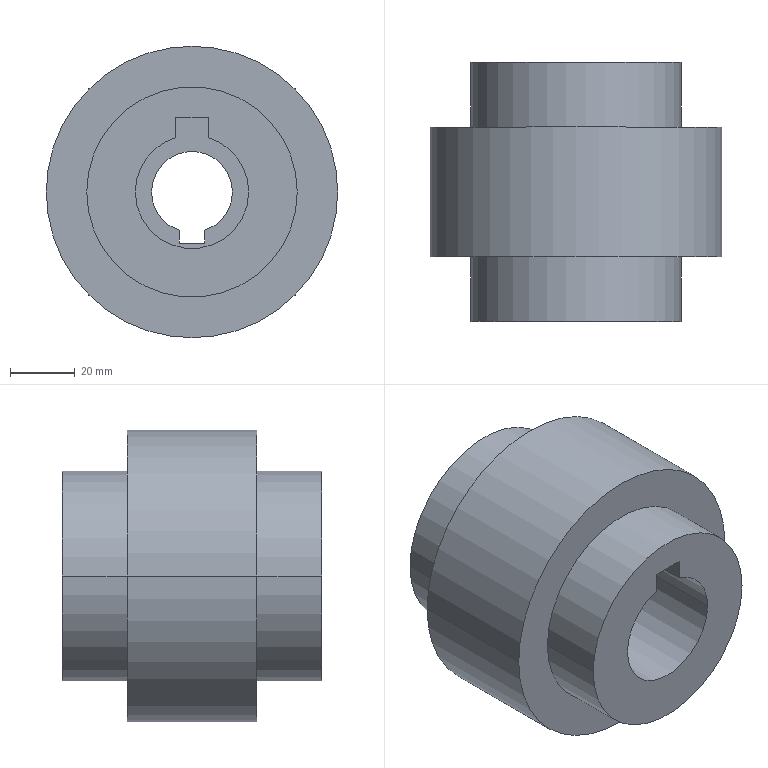Component | SolidWorks | TractorCoupling-1 | 1 solid | 23 faces | box 90 x 80 x 90 mm | volume 325660 mm3 | cylinder 12 | plane 11 | commonest cylinder face diameters 65 x4 35 x3 25 x3 90 x2
STEP:
#1=COLOUR_RGB('',0.7922,0.8196,0.9333);
#2=FILL_AREA_STYLE_COLOUR('',#1);
#3=FILL_AREA_STYLE('',(#2));
#4=SURFACE_STYLE_FILL_AREA(#3);
#5=SURFACE_SIDE_STYLE('',(#4));
#6=SURFACE_STYLE_USAGE(.BOTH.,#5);
#7=PRESENTATION_STYLE_ASSIGNMENT((#6));
#8=CARTESIAN_POINT('',(7.382,33.858,-6.811));
#9=VERTEX_POINT('',#8);
#10=CARTESIAN_POINT('',(8.76,33.858,-6.811));
#11=VERTEX_POINT('',#10);
#12=CARTESIAN_POINT('',(8.071,33.858,-6.811));
#13=DIRECTION('',(0.,-1.,0.));
#14=DIRECTION('',(1.,0.,0.));
#15=AXIS2_PLACEMENT_3D('',#12,#13,#14);
#16=CIRCLE('',#15,0.689);
#17=EDGE_CURVE('',#9,#11,#16,.T.);
#18=ORIENTED_EDGE('',*,*,#17,.F.);
#19=CARTESIAN_POINT('',(7.382,32.283,-6.811));
#20=VERTEX_POINT('',#19);
#21=CARTESIAN_POINT('',(7.382,33.858,-6.811));
#22=DIRECTION('',(0.,-1.,0.));
#23=VECTOR('',#22,39.37);
#24=LINE('',#21,#23);
#25=EDGE_CURVE('',#9,#20,#24,.T.);
#26=ORIENTED_EDGE('',*,*,#25,.T.);
#27=CARTESIAN_POINT('',(8.76,32.283,-6.811));
#28=VERTEX_POINT('',#27);
#29=CARTESIAN_POINT('',(8.071,32.283,-6.811));
#30=DIRECTION('',(0.,-1.,0.));
#31=DIRECTION('',(1.,0.,0.));
#32=AXIS2_PLACEMENT_3D('',#29,#30,#31);
#33=CIRCLE('',#32,0.689);
#34=EDGE_CURVE('',#20,#28,#33,.T.);
#35=ORIENTED_EDGE('',*,*,#34,.T.);
#36=CARTESIAN_POINT('',(8.76,33.858,-6.811));
#37=DIRECTION('',(0.,-1.,0.));
#38=VECTOR('',#37,39.37);
#39=LINE('',#36,#38);
#40=EDGE_CURVE('',#11,#28,#39,.T.);
#41=ORIENTED_EDGE('',*,*,#40,.F.);
#42=EDGE_LOOP('',(#18,#26,#35,#41));
#43=FACE_OUTER_BOUND('',#42,.T.);
#44=CARTESIAN_POINT('',(8.071,33.858,-6.811));
#45=DIRECTION('',(0.,-1.,0.));
#46=DIRECTION('',(1.,0.,0.));
#47=AXIS2_PLACEMENT_3D('',#44,#45,#46);
#48=CYLINDRICAL_SURFACE('',#47,0.689);
#49=ADVANCED_FACE('',(#43),#48,.F.);
#50=CARTESIAN_POINT('',(8.268,33.858,-6.151));
#51=VERTEX_POINT('',#50);
#52=CARTESIAN_POINT('',(8.071,33.858,-6.811));
#53=DIRECTION('',(0.,-1.,0.));
#54=DIRECTION('',(1.,0.,0.));
#55=AXIS2_PLACEMENT_3D('',#52,#53,#54);
#56=CIRCLE('',#55,0.689);
#57=EDGE_CURVE('',#11,#51,#56,.T.);
#58=ORIENTED_EDGE('',*,*,#57,.F.);
#59=ORIENTED_EDGE('',*,*,#40,.T.);
#60=CARTESIAN_POINT('',(8.268,32.283,-6.151));
#61=VERTEX_POINT('',#60);
#62=CARTESIAN_POINT('',(8.071,32.283,-6.811));
#63=DIRECTION('',(0.,-1.,0.));
#64=DIRECTION('',(1.,0.,0.));
#65=AXIS2_PLACEMENT_3D('',#62,#63,#64);
#66=CIRCLE('',#65,0.689);
#67=EDGE_CURVE('',#28,#61,#66,.T.);
#68=ORIENTED_EDGE('',*,*,#67,.T.);
#69=CARTESIAN_POINT('',(8.268,33.858,-6.151));
#70=DIRECTION('',(-0.,1.,0.));
#71=VECTOR('',#70,39.37);
#72=LINE('',#69,#71);
#73=EDGE_CURVE('',#61,#51,#72,.T.);
#74=ORIENTED_EDGE('',*,*,#73,.T.);
#75=EDGE_LOOP('',(#58,#59,#68,#74));
#76=FACE_OUTER_BOUND('',#75,.T.);
#77=CARTESIAN_POINT('',(8.071,33.858,-6.811));
#78=DIRECTION('',(0.,-1.,0.));
#79=DIRECTION('',(1.,0.,0.));
#80=AXIS2_PLACEMENT_3D('',#77,#78,#79);
#81=CYLINDRICAL_SURFACE('',#80,0.689);
#82=ADVANCED_FACE('',(#76),#81,.F.);
#83=CARTESIAN_POINT('',(6.791,32.283,-6.811));
#84=VERTEX_POINT('',#83);
#85=CARTESIAN_POINT('',(9.35,32.283,-6.811));
#86=VERTEX_POINT('',#85);
#87=CARTESIAN_POINT('',(8.071,32.283,-6.811));
#88=DIRECTION('',(0.,-1.,0.));
#89=DIRECTION('',(1.,0.,0.));
#90=AXIS2_PLACEMENT_3D('',#87,#88,#89);
#91=CIRCLE('',#90,1.28);
#92=EDGE_CURVE('',#84,#86,#91,.T.);
#93=ORIENTED_EDGE('',*,*,#92,.F.);
#94=CARTESIAN_POINT('',(6.791,33.071,-6.811));
#95=VERTEX_POINT('',#94);
#96=CARTESIAN_POINT('',(6.791,45.196,-6.811));
#97=DIRECTION('',(-0.,1.,0.));
#98=VECTOR('',#97,39.37);
#99=LINE('',#96,#98);
#100=EDGE_CURVE('',#84,#95,#99,.T.);
#101=ORIENTED_EDGE('',*,*,#100,.T.);
#102=CARTESIAN_POINT('',(9.35,33.071,-6.811));
#103=VERTEX_POINT('',#102);
#104=CARTESIAN_POINT('',(8.071,33.071,-6.811));
#105=DIRECTION('',(0.,-1.,0.));
#106=DIRECTION('',(1.,0.,0.));
#107=AXIS2_PLACEMENT_3D('',#104,#105,#106);
#108=CIRCLE('',#107,1.28);
#109=EDGE_CURVE('',#95,#103,#108,.T.);
#110=ORIENTED_EDGE('',*,*,#109,.T.);
#111=CARTESIAN_POINT('',(9.35,45.196,-6.811));
#112=DIRECTION('',(-0.,1.,0.));
#113=VECTOR('',#112,39.37);
#114=LINE('',#111,#113);
#115=EDGE_CURVE('',#86,#103,#114,.T.);
#116=ORIENTED_EDGE('',*,*,#115,.F.);
#117=EDGE_LOOP('',(#93,#101,#110,#116));
#118=FACE_OUTER_BOUND('',#117,.T.);
#119=CARTESIAN_POINT('',(8.071,45.196,-6.811));
#120=DIRECTION('',(-0.,1.,0.));
#121=DIRECTION('',(1.,0.,0.));
#122=AXIS2_PLACEMENT_3D('',#119,#120,#121);
#123=CYLINDRICAL_SURFACE('',#122,1.28);
#124=ADVANCED_FACE('',(#118),#123,.T.);
#125=CARTESIAN_POINT('',(9.35,35.433,-6.811));
#126=VERTEX_POINT('',#125);
#127=CARTESIAN_POINT('',(6.791,35.433,-6.811));
#128=VERTEX_POINT('',#127);
#129=CARTESIAN_POINT('',(8.071,35.433,-6.811));
#130=DIRECTION('',(0.,-1.,0.));
#131=DIRECTION('',(1.,0.,0.));
#132=AXIS2_PLACEMENT_3D('',#129,#130,#131);
#133=CIRCLE('',#132,1.28);
#134=EDGE_CURVE('',#126,#128,#133,.T.);
#135=ORIENTED_EDGE('',*,*,#134,.T.);
#136=CARTESIAN_POINT('',(6.791,34.646,-6.811));
#137=VERTEX_POINT('',#136);
#138=CARTESIAN_POINT('',(6.791,22.521,-6.811));
#139=DIRECTION('',(0.,-1.,0.));
#140=VECTOR('',#139,39.37);
#141=LINE('',#138,#140);
#142=EDGE_CURVE('',#128,#137,#141,.T.);
#143=ORIENTED_EDGE('',*,*,#142,.T.);
#144=CARTESIAN_POINT('',(9.35,34.646,-6.811));
#145=VERTEX_POINT('',#144);
#146=CARTESIAN_POINT('',(8.071,34.646,-6.811));
#147=DIRECTION('',(0.,-1.,0.));
#148=DIRECTION('',(1.,0.,0.));
#149=AXIS2_PLACEMENT_3D('',#146,#147,#148);
#150=CIRCLE('',#149,1.28);
#151=EDGE_CURVE('',#145,#137,#150,.T.);
#152=ORIENTED_EDGE('',*,*,#151,.F.);
#153=CARTESIAN_POINT('',(9.35,22.521,-6.811));
#154=DIRECTION('',(0.,-1.,0.));
#155=VECTOR('',#154,39.37);
#156=LINE('',#153,#155);
#157=EDGE_CURVE('',#126,#145,#156,.T.);
#158=ORIENTED_EDGE('',*,*,#157,.F.);
#159=EDGE_LOOP('',(#135,#143,#152,#158));
#160=FACE_OUTER_BOUND('',#159,.T.);
#161=CARTESIAN_POINT('',(8.071,22.521,-6.811));
#162=DIRECTION('',(0.,-1.,0.));
#163=DIRECTION('',(1.,0.,0.));
#164=AXIS2_PLACEMENT_3D('',#161,#162,#163);
#165=CYLINDRICAL_SURFACE('',#164,1.28);
#166=ADVANCED_FACE('',(#160),#165,.T.);
#167=CARTESIAN_POINT('',(9.843,34.646,-6.811));
#168=VERTEX_POINT('',#167);
#169=CARTESIAN_POINT('',(6.299,34.646,-6.811));
#170=VERTEX_POINT('',#169);
#171=CARTESIAN_POINT('',(8.071,34.646,-6.811));
#172=DIRECTION('',(0.,-1.,0.));
#173=DIRECTION('',(1.,0.,0.));
#174=AXIS2_PLACEMENT_3D('',#171,#172,#173);
#175=CIRCLE('',#174,1.772);
#176=EDGE_CURVE('',#168,#170,#175,.T.);
#177=ORIENTED_EDGE('',*,*,#176,.T.);
#178=CARTESIAN_POINT('',(6.299,33.071,-6.811));
#179=VERTEX_POINT('',#178);
#180=CARTESIAN_POINT('',(6.299,22.521,-6.811));
#181=DIRECTION('',(0.,-1.,0.));
#182=VECTOR('',#181,39.37);
#183=LINE('',#180,#182);
#184=EDGE_CURVE('',#170,#179,#183,.T.);
#185=ORIENTED_EDGE('',*,*,#184,.T.);
#186=CARTESIAN_POINT('',(9.843,33.071,-6.811));
#187=VERTEX_POINT('',#186);
#188=CARTESIAN_POINT('',(8.071,33.071,-6.811));
#189=DIRECTION('',(0.,-1.,0.));
#190=DIRECTION('',(1.,0.,0.));
#191=AXIS2_PLACEMENT_3D('',#188,#189,#190);
#192=CIRCLE('',#191,1.772);
#193=EDGE_CURVE('',#187,#179,#192,.T.);
#194=ORIENTED_EDGE('',*,*,#193,.F.);
#195=CARTESIAN_POINT('',(9.843,22.521,-6.811));
#196=DIRECTION('',(0.,-1.,0.));
#197=VECTOR('',#196,39.37);
#198=LINE('',#195,#197);
#199=EDGE_CURVE('',#168,#187,#198,.T.);
#200=ORIENTED_EDGE('',*,*,#199,.F.);
#201=EDGE_LOOP('',(#177,#185,#194,#200));
#202=FACE_OUTER_BOUND('',#201,.T.);
#203=CARTESIAN_POINT('',(8.071,22.521,-6.811));
#204=DIRECTION('',(0.,-1.,0.));
#205=DIRECTION('',(1.,0.,0.));
#206=AXIS2_PLACEMENT_3D('',#203,#204,#205);
#207=CYLINDRICAL_SURFACE('',#206,1.772);
#208=ADVANCED_FACE('',(#202),#207,.T.);
#209=CARTESIAN_POINT('',(7.579,35.433,-6.811));
#210=VERTEX_POINT('',#209);
#211=CARTESIAN_POINT('',(7.913,35.433,-7.277));
#212=VERTEX_POINT('',#211);
#213=CARTESIAN_POINT('',(8.071,35.433,-6.811));
#214=DIRECTION('',(0.,-1.,0.));
#215=DIRECTION('',(1.,0.,0.));
#216=AXIS2_PLACEMENT_3D('',#213,#214,#215);
#217=CIRCLE('',#216,0.4921);
#218=EDGE_CURVE('',#210,#212,#217,.T.);
#219=ORIENTED_EDGE('',*,*,#218,.F.);
#220=CARTESIAN_POINT('',(7.579,33.858,-6.811));
#221=VERTEX_POINT('',#220);
#222=CARTESIAN_POINT('',(7.579,22.521,-6.811));
#223=DIRECTION('',(0.,-1.,0.));
#224=VECTOR('',#223,39.37);
#225=LINE('',#222,#224);
#226=EDGE_CURVE('',#210,#221,#225,.T.);
#227=ORIENTED_EDGE('',*,*,#226,.T.);
#228=CARTESIAN_POINT('',(7.913,33.858,-7.277));
#229=VERTEX_POINT('',#228);
#230=CARTESIAN_POINT('',(8.071,33.858,-6.811));
#231=DIRECTION('',(0.,-1.,0.));
#232=DIRECTION('',(1.,0.,0.));
#233=AXIS2_PLACEMENT_3D('',#230,#231,#232);
#234=CIRCLE('',#233,0.4921);
#235=EDGE_CURVE('',#221,#229,#234,.T.);
#236=ORIENTED_EDGE('',*,*,#235,.T.);
#237=CARTESIAN_POINT('',(7.913,22.521,-7.277));
#238=DIRECTION('',(0.,-1.,0.));
#239=VECTOR('',#238,39.37);
#240=LINE('',#237,#239);
#241=EDGE_CURVE('',#212,#229,#240,.T.);
#242=ORIENTED_EDGE('',*,*,#241,.F.);
#243=EDGE_LOOP('',(#219,#227,#236,#242));
#244=FACE_OUTER_BOUND('',#243,.T.);
#245=CARTESIAN_POINT('',(8.071,22.521,-6.811));
#246=DIRECTION('',(0.,-1.,0.));
#247=DIRECTION('',(1.,0.,0.));
#248=AXIS2_PLACEMENT_3D('',#245,#246,#247);
#249=CYLINDRICAL_SURFACE('',#248,0.4921);
#250=ADVANCED_FACE('',(#244),#249,.F.);
#251=ORIENTED_EDGE('',*,*,#226,.F.);
#252=CARTESIAN_POINT('',(8.563,35.433,-6.811));
#253=VERTEX_POINT('',#252);
#254=CARTESIAN_POINT('',(8.071,35.433,-6.811));
#255=DIRECTION('',(0.,-1.,0.));
#256=DIRECTION('',(1.,0.,0.));
#257=AXIS2_PLACEMENT_3D('',#254,#255,#256);
#258=CIRCLE('',#257,0.4921);
#259=EDGE_CURVE('',#253,#210,#258,.T.);
#260=ORIENTED_EDGE('',*,*,#259,.F.);
#261=CARTESIAN_POINT('',(8.563,33.858,-6.811));
#262=VERTEX_POINT('',#261);
#263=CARTESIAN_POINT('',(8.563,22.521,-6.811));
#264=DIRECTION('',(0.,-1.,0.));
#265=VECTOR('',#264,39.37);
#266=LINE('',#263,#265);
#267=EDGE_CURVE('',#253,#262,#266,.T.);
#268=ORIENTED_EDGE('',*,*,#267,.T.);
#269=CARTESIAN_POINT('',(8.071,33.858,-6.811));
#270=DIRECTION('',(0.,-1.,0.));
#271=DIRECTION('',(1.,0.,0.));
#272=AXIS2_PLACEMENT_3D('',#269,#270,#271);
#273=CIRCLE('',#272,0.4921);
#274=EDGE_CURVE('',#262,#221,#273,.T.);
#275=ORIENTED_EDGE('',*,*,#274,.T.);
#276=EDGE_LOOP('',(#251,#260,#268,#275));
#277=FACE_OUTER_BOUND('',#276,.T.);
#278=CARTESIAN_POINT('',(8.071,22.521,-6.811));
#279=DIRECTION('',(0.,-1.,0.));
#280=DIRECTION('',(1.,0.,0.));
#281=AXIS2_PLACEMENT_3D('',#278,#279,#280);
#282=CYLINDRICAL_SURFACE('',#281,0.4921);
#283=ADVANCED_FACE('',(#277),#282,.F.);
#284=ORIENTED_EDGE('',*,*,#267,.F.);
#285=CARTESIAN_POINT('',(8.228,35.433,-7.277));
#286=VERTEX_POINT('',#285);
#287=CARTESIAN_POINT('',(8.071,35.433,-6.811));
#288=DIRECTION('',(0.,-1.,0.));
#289=DIRECTION('',(1.,0.,0.));
#290=AXIS2_PLACEMENT_3D('',#287,#288,#289);
#291=CIRCLE('',#290,0.4921);
#292=EDGE_CURVE('',#286,#253,#291,.T.);
#293=ORIENTED_EDGE('',*,*,#292,.F.);
#294=CARTESIAN_POINT('',(8.228,33.858,-7.277));
#295=VERTEX_POINT('',#294);
#296=CARTESIAN_POINT('',(8.228,22.521,-7.277));
#297=DIRECTION('',(-0.,1.,0.));
#298=VECTOR('',#297,39.37);
#299=LINE('',#296,#298);
#300=EDGE_CURVE('',#295,#286,#299,.T.);
#301=ORIENTED_EDGE('',*,*,#300,.F.);
#302=CARTESIAN_POINT('',(8.071,33.858,-6.811));
#303=DIRECTION('',(0.,-1.,0.));
#304=DIRECTION('',(1.,0.,0.));
#305=AXIS2_PLACEMENT_3D('',#302,#303,#304);
#306=CIRCLE('',#305,0.4921);
#307=EDGE_CURVE('',#295,#262,#306,.T.);
#308=ORIENTED_EDGE('',*,*,#307,.T.);
#309=EDGE_LOOP('',(#284,#293,#301,#308));
#310=FACE_OUTER_BOUND('',#309,.T.);
#311=CARTESIAN_POINT('',(8.071,22.521,-6.811));
#312=DIRECTION('',(0.,-1.,0.));
#313=DIRECTION('',(1.,0.,0.));
#314=AXIS2_PLACEMENT_3D('',#311,#312,#313);
#315=CYLINDRICAL_SURFACE('',#314,0.4921);
#316=ADVANCED_FACE('',(#310),#315,.F.);
#317=ORIENTED_EDGE('',*,*,#184,.F.);
#318=CARTESIAN_POINT('',(8.071,34.646,-6.811));
#319=DIRECTION('',(0.,-1.,0.));
#320=DIRECTION('',(1.,0.,0.));
#321=AXIS2_PLACEMENT_3D('',#318,#319,#320);
#322=CIRCLE('',#321,1.772);
#323=EDGE_CURVE('',#170,#168,#322,.T.);
#324=ORIENTED_EDGE('',*,*,#323,.T.);
#325=ORIENTED_EDGE('',*,*,#199,.T.);
#326=CARTESIAN_POINT('',(8.071,33.071,-6.811));
#327=DIRECTION('',(0.,-1.,0.));
#328=DIRECTION('',(1.,0.,0.));
#329=AXIS2_PLACEMENT_3D('',#326,#327,#328);
#330=CIRCLE('',#329,1.772);
#331=EDGE_CURVE('',#179,#187,#330,.T.);
#332=ORIENTED_EDGE('',*,*,#331,.F.);
#333=EDGE_LOOP('',(#317,#324,#325,#332));
#334=FACE_OUTER_BOUND('',#333,.T.);
#335=CARTESIAN_POINT('',(8.071,22.521,-6.811));
#336=DIRECTION('',(0.,-1.,0.));
#337=DIRECTION('',(1.,0.,0.));
#338=AXIS2_PLACEMENT_3D('',#335,#336,#337);
#339=CYLINDRICAL_SURFACE('',#338,1.772);
#340=ADVANCED_FACE('',(#334),#339,.T.);
#341=ORIENTED_EDGE('',*,*,#151,.T.);
#342=CARTESIAN_POINT('',(8.071,34.646,-6.811));
#343=DIRECTION('',(0.,-1.,0.));
#344=DIRECTION('',(1.,0.,0.));
#345=AXIS2_PLACEMENT_3D('',#342,#343,#344);
#346=CIRCLE('',#345,1.28);
#347=EDGE_CURVE('',#137,#145,#346,.T.);
#348=ORIENTED_EDGE('',*,*,#347,.T.);
#349=EDGE_LOOP('',(#341,#348));
#350=FACE_BOUND('',#349,.T.);
#351=ORIENTED_EDGE('',*,*,#176,.F.);
#352=ORIENTED_EDGE('',*,*,#323,.F.);
#353=EDGE_LOOP('',(#351,#352));
#354=FACE_OUTER_BOUND('',#353,.T.);
#355=CARTESIAN_POINT('',(9.843,34.646,-6.811));
#356=DIRECTION('',(-0.,1.,0.));
#357=DIRECTION('',(-1.,-0.,0.));
#358=AXIS2_PLACEMENT_3D('',#355,#356,#357);
#359=PLANE('',#358);
#360=ADVANCED_FACE('',(#350,#354),#359,.T.);
#361=ORIENTED_EDGE('',*,*,#142,.F.);
#362=CARTESIAN_POINT('',(8.071,35.433,-6.811));
#363=DIRECTION('',(0.,-1.,0.));
#364=DIRECTION('',(1.,0.,0.));
#365=AXIS2_PLACEMENT_3D('',#362,#363,#364);
#366=CIRCLE('',#365,1.28);
#367=EDGE_CURVE('',#128,#126,#366,.T.);
#368=ORIENTED_EDGE('',*,*,#367,.T.);
#369=ORIENTED_EDGE('',*,*,#157,.T.);
#370=ORIENTED_EDGE('',*,*,#347,.F.);
#371=EDGE_LOOP('',(#361,#368,#369,#370));
#372=FACE_OUTER_BOUND('',#371,.T.);
#373=CARTESIAN_POINT('',(8.071,22.521,-6.811));
#374=DIRECTION('',(0.,-1.,0.));
#375=DIRECTION('',(1.,0.,0.));
#376=AXIS2_PLACEMENT_3D('',#373,#374,#375);
#377=CYLINDRICAL_SURFACE('',#376,1.28);
#378=ADVANCED_FACE('',(#372),#377,.T.);
#379=CARTESIAN_POINT('',(7.913,35.433,-7.433));
#380=VERTEX_POINT('',#379);
#381=CARTESIAN_POINT('',(7.913,35.433,-7.433));
#382=DIRECTION('',(0.,0.,1.));
#383=VECTOR('',#382,39.37);
#384=LINE('',#381,#383);
#385=EDGE_CURVE('',#380,#212,#384,.T.);
#386=ORIENTED_EDGE('',*,*,#385,.F.);
#387=CARTESIAN_POINT('',(8.228,35.433,-7.433));
#388=VERTEX_POINT('',#387);
#389=CARTESIAN_POINT('',(7.913,35.433,-7.433));
#390=DIRECTION('',(-1.,-0.,0.));
#391=VECTOR('',#390,39.37);
#392=LINE('',#389,#391);
#393=EDGE_CURVE('',#388,#380,#392,.T.);
#394=ORIENTED_EDGE('',*,*,#393,.F.);
#395=CARTESIAN_POINT('',(8.228,35.433,-7.433));
#396=DIRECTION('',(-0.,0.,-1.));
#397=VECTOR('',#396,39.37);
#398=LINE('',#395,#397);
#399=EDGE_CURVE('',#286,#388,#398,.T.);
#400=ORIENTED_EDGE('',*,*,#399,.F.);
#401=ORIENTED_EDGE('',*,*,#292,.T.);
#402=ORIENTED_EDGE('',*,*,#259,.T.);
#403=ORIENTED_EDGE('',*,*,#218,.T.);
#404=EDGE_LOOP('',(#386,#394,#400,#401,#402,#403));
#405=FACE_BOUND('',#404,.T.);
#406=ORIENTED_EDGE('',*,*,#134,.F.);
#407=ORIENTED_EDGE('',*,*,#367,.F.);
#408=EDGE_LOOP('',(#406,#407));
#409=FACE_OUTER_BOUND('',#408,.T.);
#410=CARTESIAN_POINT('',(9.35,35.433,-6.811));
#411=DIRECTION('',(-0.,1.,0.));
#412=DIRECTION('',(-1.,-0.,0.));
#413=AXIS2_PLACEMENT_3D('',#410,#411,#412);
#414=PLANE('',#413);
#415=ADVANCED_FACE('',(#405,#409),#414,.T.);
#416=CARTESIAN_POINT('',(8.071,33.071,-6.811));
#417=DIRECTION('',(0.,-1.,0.));
#418=DIRECTION('',(1.,0.,0.));
#419=AXIS2_PLACEMENT_3D('',#416,#417,#418);
#420=CIRCLE('',#419,1.28);
#421=EDGE_CURVE('',#103,#95,#420,.T.);
#422=ORIENTED_EDGE('',*,*,#421,.F.);
#423=ORIENTED_EDGE('',*,*,#109,.F.);
#424=EDGE_LOOP('',(#422,#423));
#425=FACE_BOUND('',#424,.T.);
#426=ORIENTED_EDGE('',*,*,#193,.T.);
#427=ORIENTED_EDGE('',*,*,#331,.T.);
#428=EDGE_LOOP('',(#426,#427));
#429=FACE_OUTER_BOUND('',#428,.T.);
#430=CARTESIAN_POINT('',(9.843,33.071,-6.811));
#431=DIRECTION('',(0.,-1.,0.));
#432=DIRECTION('',(-1.,-0.,0.));
#433=AXIS2_PLACEMENT_3D('',#430,#431,#432);
#434=PLANE('',#433);
#435=ADVANCED_FACE('',(#425,#429),#434,.T.);
#436=ORIENTED_EDGE('',*,*,#100,.F.);
#437=CARTESIAN_POINT('',(8.071,32.283,-6.811));
#438=DIRECTION('',(0.,-1.,0.));
#439=DIRECTION('',(1.,0.,0.));
#440=AXIS2_PLACEMENT_3D('',#437,#438,#439);
#441=CIRCLE('',#440,1.28);
#442=EDGE_CURVE('',#86,#84,#441,.T.);
#443=ORIENTED_EDGE('',*,*,#442,.F.);
#444=ORIENTED_EDGE('',*,*,#115,.T.);
#445=ORIENTED_EDGE('',*,*,#421,.T.);
#446=EDGE_LOOP('',(#436,#443,#444,#445));
#447=FACE_OUTER_BOUND('',#446,.T.);
#448=CARTESIAN_POINT('',(8.071,45.196,-6.811));
#449=DIRECTION('',(-0.,1.,0.));
#450=DIRECTION('',(1.,0.,0.));
#451=AXIS2_PLACEMENT_3D('',#448,#449,#450);
#452=CYLINDRICAL_SURFACE('',#451,1.28);
#453=ADVANCED_FACE('',(#447),#452,.T.);
#454=CARTESIAN_POINT('',(7.874,32.283,-5.906));
#455=VERTEX_POINT('',#454);
#456=CARTESIAN_POINT('',(7.874,32.283,-6.151));
#457=VERTEX_POINT('',#456);
#458=CARTESIAN_POINT('',(7.874,32.283,-5.906));
#459=DIRECTION('',(0.,0.,-1.));
#460=VECTOR('',#459,39.37);
#461=LINE('',#458,#460);
#462=EDGE_CURVE('',#455,#457,#461,.T.);
#463=ORIENTED_EDGE('',*,*,#462,.F.);
#464=CARTESIAN_POINT('',(8.268,32.283,-5.906));
#465=VERTEX_POINT('',#464);
#466=CARTESIAN_POINT('',(7.874,32.283,-5.906));
#467=DIRECTION('',(-1.,-0.,0.));
#468=VECTOR('',#467,39.37);
#469=LINE('',#466,#468);
#470=EDGE_CURVE('',#465,#455,#469,.T.);
#471=ORIENTED_EDGE('',*,*,#470,.F.);
#472=CARTESIAN_POINT('',(8.268,32.283,-5.906));
#473=DIRECTION('',(-0.,0.,1.));
#474=VECTOR('',#473,39.37);
#475=LINE('',#472,#474);
#476=EDGE_CURVE('',#61,#465,#475,.T.);
#477=ORIENTED_EDGE('',*,*,#476,.F.);
#478=ORIENTED_EDGE('',*,*,#67,.F.);
#479=ORIENTED_EDGE('',*,*,#34,.F.);
#480=CARTESIAN_POINT('',(8.071,32.283,-6.811));
#481=DIRECTION('',(0.,-1.,0.));
#482=DIRECTION('',(1.,0.,0.));
#483=AXIS2_PLACEMENT_3D('',#480,#481,#482);
#484=CIRCLE('',#483,0.689);
#485=EDGE_CURVE('',#457,#20,#484,.T.);
#486=ORIENTED_EDGE('',*,*,#485,.F.);
#487=EDGE_LOOP('',(#463,#471,#477,#478,#479,#486));
#488=FACE_BOUND('',#487,.T.);
#489=ORIENTED_EDGE('',*,*,#442,.T.);
#490=ORIENTED_EDGE('',*,*,#92,.T.);
#491=EDGE_LOOP('',(#489,#490));
#492=FACE_OUTER_BOUND('',#491,.T.);
#493=CARTESIAN_POINT('',(9.35,32.283,-6.811));
#494=DIRECTION('',(0.,-1.,0.));
#495=DIRECTION('',(-1.,-0.,0.));
#496=AXIS2_PLACEMENT_3D('',#493,#494,#495);
#497=PLANE('',#496);
#498=ADVANCED_FACE('',(#488,#492),#497,.T.);
#499=ORIENTED_EDGE('',*,*,#25,.F.);
#500=CARTESIAN_POINT('',(7.874,33.858,-6.151));
#501=VERTEX_POINT('',#500);
#502=CARTESIAN_POINT('',(8.071,33.858,-6.811));
#503=DIRECTION('',(0.,-1.,0.));
#504=DIRECTION('',(1.,0.,0.));
#505=AXIS2_PLACEMENT_3D('',#502,#503,#504);
#506=CIRCLE('',#505,0.689);
#507=EDGE_CURVE('',#501,#9,#506,.T.);
#508=ORIENTED_EDGE('',*,*,#507,.F.);
#509=CARTESIAN_POINT('',(7.874,33.858,-6.151));
#510=DIRECTION('',(0.,-1.,0.));
#511=VECTOR('',#510,39.37);
#512=LINE('',#509,#511);
#513=EDGE_CURVE('',#501,#457,#512,.T.);
#514=ORIENTED_EDGE('',*,*,#513,.T.);
#515=ORIENTED_EDGE('',*,*,#485,.T.);
#516=EDGE_LOOP('',(#499,#508,#514,#515));
#517=FACE_OUTER_BOUND('',#516,.T.);
#518=CARTESIAN_POINT('',(8.071,33.858,-6.811));
#519=DIRECTION('',(0.,-1.,0.));
#520=DIRECTION('',(1.,0.,0.));
#521=AXIS2_PLACEMENT_3D('',#518,#519,#520);
#522=CYLINDRICAL_SURFACE('',#521,0.689);
#523=ADVANCED_FACE('',(#517),#522,.F.);
#524=CARTESIAN_POINT('',(7.913,33.858,-7.433));
#525=VERTEX_POINT('',#524);
#526=CARTESIAN_POINT('',(7.913,33.858,-7.433));
#527=DIRECTION('',(0.,0.,1.));
#528=VECTOR('',#527,39.37);
#529=LINE('',#526,#528);
#530=EDGE_CURVE('',#525,#229,#529,.T.);
#531=ORIENTED_EDGE('',*,*,#530,.T.);
#532=ORIENTED_EDGE('',*,*,#235,.F.);
#533=ORIENTED_EDGE('',*,*,#274,.F.);
#534=ORIENTED_EDGE('',*,*,#307,.F.);
#535=CARTESIAN_POINT('',(8.228,33.858,-7.433));
#536=VERTEX_POINT('',#535);
#537=CARTESIAN_POINT('',(8.228,33.858,-6.811));
#538=DIRECTION('',(0.,0.,1.));
#539=VECTOR('',#538,39.37);
#540=LINE('',#537,#539);
#541=EDGE_CURVE('',#536,#295,#540,.T.);
#542=ORIENTED_EDGE('',*,*,#541,.F.);
#543=CARTESIAN_POINT('',(7.913,33.858,-7.433));
#544=DIRECTION('',(-1.,-0.,0.));
#545=VECTOR('',#544,39.37);
#546=LINE('',#543,#545);
#547=EDGE_CURVE('',#536,#525,#546,.T.);
#548=ORIENTED_EDGE('',*,*,#547,.T.);
#549=EDGE_LOOP('',(#531,#532,#533,#534,#542,#548));
#550=FACE_BOUND('',#549,.T.);
#551=ORIENTED_EDGE('',*,*,#507,.T.);
#552=ORIENTED_EDGE('',*,*,#17,.T.);
#553=ORIENTED_EDGE('',*,*,#57,.T.);
#554=CARTESIAN_POINT('',(8.268,33.858,-5.906));
#555=VERTEX_POINT('',#554);
#556=CARTESIAN_POINT('',(8.268,33.858,-5.906));
#557=DIRECTION('',(-0.,0.,1.));
#558=VECTOR('',#557,39.37);
#559=LINE('',#556,#558);
#560=EDGE_CURVE('',#51,#555,#559,.T.);
#561=ORIENTED_EDGE('',*,*,#560,.T.);
#562=CARTESIAN_POINT('',(7.874,33.858,-5.906));
#563=VERTEX_POINT('',#562);
#564=CARTESIAN_POINT('',(7.874,33.858,-5.906));
#565=DIRECTION('',(-1.,-0.,0.));
#566=VECTOR('',#565,39.37);
#567=LINE('',#564,#566);
#568=EDGE_CURVE('',#555,#563,#567,.T.);
#569=ORIENTED_EDGE('',*,*,#568,.T.);
#570=CARTESIAN_POINT('',(7.874,33.858,-5.906));
#571=DIRECTION('',(0.,0.,-1.));
#572=VECTOR('',#571,39.37);
#573=LINE('',#570,#572);
#574=EDGE_CURVE('',#563,#501,#573,.T.);
#575=ORIENTED_EDGE('',*,*,#574,.T.);
#576=EDGE_LOOP('',(#551,#552,#553,#561,#569,#575));
#577=FACE_OUTER_BOUND('',#576,.T.);
#578=CARTESIAN_POINT('',(8.071,33.858,-6.811));
#579=DIRECTION('',(0.,-1.,0.));
#580=DIRECTION('',(1.,0.,0.));
#581=AXIS2_PLACEMENT_3D('',#578,#579,#580);
#582=PLANE('',#581);
#583=ADVANCED_FACE('',(#550,#577),#582,.T.);
#584=ORIENTED_EDGE('',*,*,#574,.F.);
#585=CARTESIAN_POINT('',(7.874,33.858,-5.906));
#586=DIRECTION('',(0.,-1.,0.));
#587=VECTOR('',#586,39.37);
#588=LINE('',#585,#587);
#589=EDGE_CURVE('',#563,#455,#588,.T.);
#590=ORIENTED_EDGE('',*,*,#589,.T.);
#591=ORIENTED_EDGE('',*,*,#462,.T.);
#592=ORIENTED_EDGE('',*,*,#513,.F.);
#593=EDGE_LOOP('',(#584,#590,#591,#592));
#594=FACE_OUTER_BOUND('',#593,.T.);
#595=CARTESIAN_POINT('',(7.874,33.858,-5.906));
#596=DIRECTION('',(-1.,-0.,-0.));
#597=DIRECTION('',(0.,-1.,0.));
#598=AXIS2_PLACEMENT_3D('',#595,#596,#597);
#599=PLANE('',#598);
#600=ADVANCED_FACE('',(#594),#599,.F.);
#601=ORIENTED_EDGE('',*,*,#476,.T.);
#602=CARTESIAN_POINT('',(8.268,33.858,-5.906));
#603=DIRECTION('',(0.,-1.,0.));
#604=VECTOR('',#603,39.37);
#605=LINE('',#602,#604);
#606=EDGE_CURVE('',#555,#465,#605,.T.);
#607=ORIENTED_EDGE('',*,*,#606,.F.);
#608=ORIENTED_EDGE('',*,*,#560,.F.);
#609=ORIENTED_EDGE('',*,*,#73,.F.);
#610=EDGE_LOOP('',(#601,#607,#608,#609));
#611=FACE_OUTER_BOUND('',#610,.T.);
#612=CARTESIAN_POINT('',(8.268,33.858,-5.906));
#613=DIRECTION('',(1.,0.,0.));
#614=DIRECTION('',(-0.,1.,0.));
#615=AXIS2_PLACEMENT_3D('',#612,#613,#614);
#616=PLANE('',#615);
#617=ADVANCED_FACE('',(#611),#616,.F.);
#618=ORIENTED_EDGE('',*,*,#470,.T.);
#619=ORIENTED_EDGE('',*,*,#589,.F.);
#620=ORIENTED_EDGE('',*,*,#568,.F.);
#621=ORIENTED_EDGE('',*,*,#606,.T.);
#622=EDGE_LOOP('',(#618,#619,#620,#621));
#623=FACE_OUTER_BOUND('',#622,.T.);
#624=CARTESIAN_POINT('',(7.874,33.858,-5.906));
#625=DIRECTION('',(0.,0.,1.));
#626=DIRECTION('',(1.,0.,0.));
#627=AXIS2_PLACEMENT_3D('',#624,#625,#626);
#628=PLANE('',#627);
#629=ADVANCED_FACE('',(#623),#628,.F.);
#630=ORIENTED_EDGE('',*,*,#241,.T.);
#631=ORIENTED_EDGE('',*,*,#530,.F.);
#632=CARTESIAN_POINT('',(7.913,33.858,-7.433));
#633=DIRECTION('',(-0.,1.,0.));
#634=VECTOR('',#633,39.37);
#635=LINE('',#632,#634);
#636=EDGE_CURVE('',#525,#380,#635,.T.);
#637=ORIENTED_EDGE('',*,*,#636,.T.);
#638=ORIENTED_EDGE('',*,*,#385,.T.);
#639=EDGE_LOOP('',(#630,#631,#637,#638));
#640=FACE_OUTER_BOUND('',#639,.T.);
#641=CARTESIAN_POINT('',(7.913,33.858,-7.433));
#642=DIRECTION('',(-1.,-0.,0.));
#643=DIRECTION('',(0.,-1.,0.));
#644=AXIS2_PLACEMENT_3D('',#641,#642,#643);
#645=PLANE('',#644);
#646=ADVANCED_FACE('',(#640),#645,.F.);
#647=ORIENTED_EDGE('',*,*,#393,.T.);
#648=ORIENTED_EDGE('',*,*,#636,.F.);
#649=ORIENTED_EDGE('',*,*,#547,.F.);
#650=CARTESIAN_POINT('',(8.228,33.858,-7.433));
#651=DIRECTION('',(-0.,1.,0.));
#652=VECTOR('',#651,39.37);
#653=LINE('',#650,#652);
#654=EDGE_CURVE('',#536,#388,#653,.T.);
#655=ORIENTED_EDGE('',*,*,#654,.T.);
#656=EDGE_LOOP('',(#647,#648,#649,#655));
#657=FACE_OUTER_BOUND('',#656,.T.);
#658=CARTESIAN_POINT('',(7.913,33.858,-7.433));
#659=DIRECTION('',(0.,0.,-1.));
#660=DIRECTION('',(-1.,0.,0.));
#661=AXIS2_PLACEMENT_3D('',#658,#659,#660);
#662=PLANE('',#661);
#663=ADVANCED_FACE('',(#657),#662,.F.);
#664=ORIENTED_EDGE('',*,*,#300,.T.);
#665=ORIENTED_EDGE('',*,*,#399,.T.);
#666=ORIENTED_EDGE('',*,*,#654,.F.);
#667=ORIENTED_EDGE('',*,*,#541,.T.);
#668=EDGE_LOOP('',(#664,#665,#666,#667));
#669=FACE_OUTER_BOUND('',#668,.T.);
#670=CARTESIAN_POINT('',(8.228,33.858,-7.433));
#671=DIRECTION('',(1.,0.,-0.));
#672=DIRECTION('',(-0.,1.,0.));
#673=AXIS2_PLACEMENT_3D('',#670,#671,#672);
#674=PLANE('',#673);
#675=ADVANCED_FACE('',(#669),#674,.F.);
#676=CLOSED_SHELL('',(#49,#82,#124,#166,#208,#250,#283,#316,#340,#360,#378,#415,#435,#453,#498,#523,#583,#600,#617,#629,#646,#663,#675));
#677=MANIFOLD_SOLID_BREP('',#676);
#678=STYLED_ITEM('',(#7),#677);
#679=(LENGTH_UNIT()NAMED_UNIT(*)SI_UNIT($,.METRE.));
#680=LENGTH_MEASURE_WITH_UNIT(LENGTH_MEASURE(0.0254),#679);
#681=DIMENSIONAL_EXPONENTS(1.,0.,0.,0.,0.,0.,0.);
#682=(CONVERSION_BASED_UNIT('',#680)LENGTH_UNIT()NAMED_UNIT(#681));
#683=UNCERTAINTY_MEASURE_WITH_UNIT(LENGTH_MEASURE(0.00001),#682,'','');
#684=(NAMED_UNIT(*)PLANE_ANGLE_UNIT()SI_UNIT($,.RADIAN.));
#685=(NAMED_UNIT(*)SI_UNIT($,.STERADIAN.)SOLID_ANGLE_UNIT());
#686=(GEOMETRIC_REPRESENTATION_CONTEXT(3)GLOBAL_UNCERTAINTY_ASSIGNED_CONTEXT((#683))GLOBAL_UNIT_ASSIGNED_CONTEXT((#682,#684,#685))REPRESENTATION_CONTEXT('',''));
#687=MECHANICAL_DESIGN_GEOMETRIC_PRESENTATION_REPRESENTATION('',(#678),#686);
#688=CARTESIAN_POINT('',(0.,0.,0.));
#689=DIRECTION('',(0.,0.,1.));
#690=DIRECTION('',(1.,0.,0.));
#691=AXIS2_PLACEMENT_3D('',#688,#689,#690);
#692=(LENGTH_UNIT()NAMED_UNIT(*)SI_UNIT($,.METRE.));
#693=LENGTH_MEASURE_WITH_UNIT(LENGTH_MEASURE(0.0254),#692);
#694=DIMENSIONAL_EXPONENTS(1.,0.,0.,0.,0.,0.,0.);
#695=(CONVERSION_BASED_UNIT('',#693)LENGTH_UNIT()NAMED_UNIT(#694));
#696=UNCERTAINTY_MEASURE_WITH_UNIT(LENGTH_MEASURE(0.00001),#695,'','');
#697=(NAMED_UNIT(*)PLANE_ANGLE_UNIT()SI_UNIT($,.RADIAN.));
#698=(NAMED_UNIT(*)SI_UNIT($,.STERADIAN.)SOLID_ANGLE_UNIT());
#699=(GEOMETRIC_REPRESENTATION_CONTEXT(3)GLOBAL_UNCERTAINTY_ASSIGNED_CONTEXT((#696))GLOBAL_UNIT_ASSIGNED_CONTEXT((#695,#697,#698))REPRESENTATION_CONTEXT('',''));
#700=ADVANCED_BREP_SHAPE_REPRESENTATION('',(#677,#691),#699);
#701=PRESENTATION_LAYER_ASSIGNMENT('','',(#678));